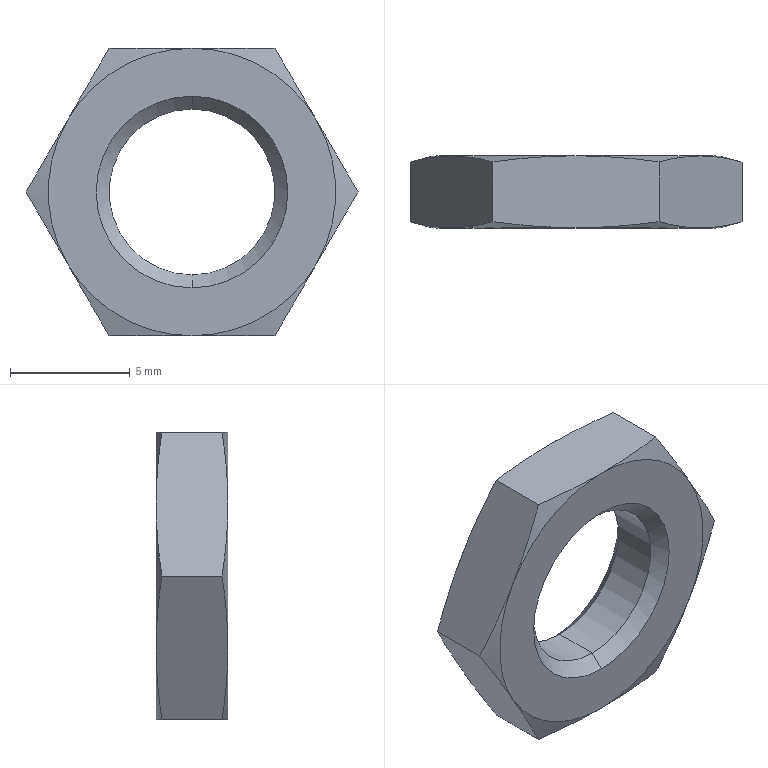Component | SolidWorks | ZPT06UNK6_B5_A80214-1_ZPT2_8_B_NUT0214-1 | 1 solid | 26 faces | box 13.86 x 3 x 12 mm | volume 253 mm3 | cone 16 | plane 8 | cylinder 2 | commonest cylinder face diameters 6.917 x2
build123d program:
from build123d import *

# Parameters (mm, degrees)
CUT_EXTRUDE1_DEPTH      = 1.5
CUT_EXTRUDE1_DEPTH_BACK = 1.5
SKETCH2_R               = 12


with BuildPart() as part:
    # Sketch1 → Revolve1 (revolve)
    with BuildSketch(Plane.XY, mode=Mode.PRIVATE) as revolve1_sk:
        Polygon((3.458, -0.9585), (4, -1.5), (6, -1.5), (9.6, -0.5354), (9.6, 0.5354), (6, 1.5), (4, 1.5), (3.458, 0.9585), align=None)
    revolve(revolve1_sk.sketch.rotate(Axis((0, -1.5, 0), (0, 1, 0)), 270), axis=Axis((0, -1.5, 0), (0, 1, 0)))

    # Sketch2 → Cut-Extrude1 (cut, two sides: drawn at the far end of the back side and taken through both)
    with BuildSketch(Plane(origin=(0, 0, 0), x_dir=(1, 0, 0), z_dir=(0, 1, 0)).offset(-CUT_EXTRUDE1_DEPTH_BACK)):
        Circle(SKETCH2_R)
        Polygon((-6.928, 0), (-3.464, -6), (3.464, -6), (6.928, 0), (3.464, 6), (-3.464, 6), align=None, mode=Mode.SUBTRACT)
    extrude(amount=CUT_EXTRUDE1_DEPTH + CUT_EXTRUDE1_DEPTH_BACK, mode=Mode.SUBTRACT)


solid = part.part

# Placed as in the assembly
solid = solid.moved(Location((-75, -53, 9.1), (0, 0, 0)))
STEP:
#1=CARTESIAN_POINT('',(-2.953,-2.049,0.2221));
#2=VERTEX_POINT('',#1);
#3=CARTESIAN_POINT('',(-2.953,-2.049,0.4944));
#4=VERTEX_POINT('',#3);
#5=CARTESIAN_POINT('',(-2.953,-2.049,0.3583));
#6=DIRECTION('',(0.,1.,0.));
#7=DIRECTION('',(0.,0.,1.));
#8=AXIS2_PLACEMENT_3D('',#5,#6,#7);
#9=CIRCLE('',#8,0.1362);
#10=EDGE_CURVE('',#2,#4,#9,.T.);
#11=ORIENTED_EDGE('',*,*,#10,.F.);
#12=CARTESIAN_POINT('',(-2.953,-2.028,0.2008));
#13=VERTEX_POINT('',#12);
#14=CARTESIAN_POINT('',(-2.953,-2.028,0.2008));
#15=DIRECTION('',(0.,0.7071,-0.7071));
#16=VECTOR('',#15,39.37);
#17=LINE('',#14,#16);
#18=EDGE_CURVE('',#2,#13,#17,.T.);
#19=ORIENTED_EDGE('',*,*,#18,.T.);
#20=CARTESIAN_POINT('',(-2.953,-2.028,0.5157));
#21=VERTEX_POINT('',#20);
#22=CARTESIAN_POINT('',(-2.953,-2.028,0.3583));
#23=DIRECTION('',(0.,1.,0.));
#24=DIRECTION('',(0.,0.,1.));
#25=AXIS2_PLACEMENT_3D('',#22,#23,#24);
#26=CIRCLE('',#25,0.1575);
#27=EDGE_CURVE('',#13,#21,#26,.T.);
#28=ORIENTED_EDGE('',*,*,#27,.T.);
#29=CARTESIAN_POINT('',(-2.953,-2.028,0.5157));
#30=DIRECTION('',(0.,0.7071,0.7071));
#31=VECTOR('',#30,39.37);
#32=LINE('',#29,#31);
#33=EDGE_CURVE('',#4,#21,#32,.T.);
#34=ORIENTED_EDGE('',*,*,#33,.F.);
#35=EDGE_LOOP('',(#11,#19,#28,#34));
#36=FACE_OUTER_BOUND('',#35,.T.);
#37=CARTESIAN_POINT('',(-2.953,-2.028,0.3583));
#38=DIRECTION('',(0.,1.,0.));
#39=DIRECTION('',(0.,0.,1.));
#40=AXIS2_PLACEMENT_3D('',#37,#38,#39);
#41=CONICAL_SURFACE('',#40,0.1575,0.7854);
#42=ADVANCED_FACE('',(#36),#41,.F.);
#43=CARTESIAN_POINT('',(-2.953,-2.124,0.2221));
#44=VERTEX_POINT('',#43);
#45=CARTESIAN_POINT('',(-2.953,-2.124,0.4944));
#46=VERTEX_POINT('',#45);
#47=CARTESIAN_POINT('',(-2.953,-2.124,0.3583));
#48=DIRECTION('',(0.,1.,0.));
#49=DIRECTION('',(0.,0.,1.));
#50=AXIS2_PLACEMENT_3D('',#47,#48,#49);
#51=CIRCLE('',#50,0.1362);
#52=EDGE_CURVE('',#44,#46,#51,.T.);
#53=ORIENTED_EDGE('',*,*,#52,.T.);
#54=CARTESIAN_POINT('',(-2.953,-2.146,0.5157));
#55=VERTEX_POINT('',#54);
#56=CARTESIAN_POINT('',(-2.953,-2.124,0.4944));
#57=DIRECTION('',(0.,-0.7071,0.7071));
#58=VECTOR('',#57,39.37);
#59=LINE('',#56,#58);
#60=EDGE_CURVE('',#46,#55,#59,.T.);
#61=ORIENTED_EDGE('',*,*,#60,.T.);
#62=CARTESIAN_POINT('',(-2.953,-2.146,0.2008));
#63=VERTEX_POINT('',#62);
#64=CARTESIAN_POINT('',(-2.953,-2.146,0.3583));
#65=DIRECTION('',(0.,1.,0.));
#66=DIRECTION('',(0.,0.,1.));
#67=AXIS2_PLACEMENT_3D('',#64,#65,#66);
#68=CIRCLE('',#67,0.1575);
#69=EDGE_CURVE('',#63,#55,#68,.T.);
#70=ORIENTED_EDGE('',*,*,#69,.F.);
#71=CARTESIAN_POINT('',(-2.953,-2.124,0.2221));
#72=DIRECTION('',(0.,-0.7071,-0.7071));
#73=VECTOR('',#72,39.37);
#74=LINE('',#71,#73);
#75=EDGE_CURVE('',#44,#63,#74,.T.);
#76=ORIENTED_EDGE('',*,*,#75,.F.);
#77=EDGE_LOOP('',(#53,#61,#70,#76));
#78=FACE_OUTER_BOUND('',#77,.T.);
#79=CARTESIAN_POINT('',(-2.953,-2.124,0.3583));
#80=DIRECTION('',(0.,-1.,0.));
#81=DIRECTION('',(0.,0.,-1.));
#82=AXIS2_PLACEMENT_3D('',#79,#80,#81);
#83=CONICAL_SURFACE('',#82,0.1362,0.7854);
#84=ADVANCED_FACE('',(#78),#83,.F.);
#85=ORIENTED_EDGE('',*,*,#52,.F.);
#86=CARTESIAN_POINT('',(-2.953,-2.146,0.2221));
#87=DIRECTION('',(0.,1.,0.));
#88=VECTOR('',#87,39.37);
#89=LINE('',#86,#88);
#90=EDGE_CURVE('',#44,#2,#89,.T.);
#91=ORIENTED_EDGE('',*,*,#90,.T.);
#92=ORIENTED_EDGE('',*,*,#10,.T.);
#93=CARTESIAN_POINT('',(-2.953,-2.146,0.4944));
#94=DIRECTION('',(0.,1.,0.));
#95=VECTOR('',#94,39.37);
#96=LINE('',#93,#95);
#97=EDGE_CURVE('',#46,#4,#96,.T.);
#98=ORIENTED_EDGE('',*,*,#97,.F.);
#99=EDGE_LOOP('',(#85,#91,#92,#98));
#100=FACE_OUTER_BOUND('',#99,.T.);
#101=CARTESIAN_POINT('',(-2.953,-2.146,0.3583));
#102=DIRECTION('',(0.,1.,0.));
#103=DIRECTION('',(0.,0.,1.));
#104=AXIS2_PLACEMENT_3D('',#101,#102,#103);
#105=CYLINDRICAL_SURFACE('',#104,0.1362);
#106=ADVANCED_FACE('',(#100),#105,.F.);
#107=CARTESIAN_POINT('',(-2.68,-2.136,0.3583));
#108=VERTEX_POINT('',#107);
#109=CARTESIAN_POINT('',(-2.748,-2.146,0.2402));
#110=VERTEX_POINT('',#109);
#111=CARTESIAN_POINT('',(-2.68,-2.136,0.3583));
#112=CARTESIAN_POINT('',(-2.703,-2.142,0.3189));
#113=CARTESIAN_POINT('',(-2.725,-2.146,0.2795));
#114=CARTESIAN_POINT('',(-2.748,-2.146,0.2402));
#115=B_SPLINE_CURVE_WITH_KNOTS('',3,(#111,#112,#113,#114),.UNSPECIFIED.,.F.,.F.,(4,4),(0.00000023,0.003464),.UNSPECIFIED.);
#116=EDGE_CURVE('',#108,#110,#115,.T.);
#117=ORIENTED_EDGE('',*,*,#116,.F.);
#118=CARTESIAN_POINT('',(-2.748,-2.146,0.4764));
#119=VERTEX_POINT('',#118);
#120=CARTESIAN_POINT('',(-2.748,-2.146,0.4764));
#121=CARTESIAN_POINT('',(-2.725,-2.146,0.437));
#122=CARTESIAN_POINT('',(-2.703,-2.142,0.3976));
#123=CARTESIAN_POINT('',(-2.68,-2.136,0.3583));
#124=B_SPLINE_CURVE_WITH_KNOTS('',3,(#120,#121,#122,#123),.UNSPECIFIED.,.F.,.F.,(4,4),(0.003464,0.006928),.UNSPECIFIED.);
#125=EDGE_CURVE('',#119,#108,#124,.T.);
#126=ORIENTED_EDGE('',*,*,#125,.F.);
#127=CARTESIAN_POINT('',(-2.953,-2.146,0.3583));
#128=DIRECTION('',(0.,1.,0.));
#129=DIRECTION('',(0.,0.,1.));
#130=AXIS2_PLACEMENT_3D('',#127,#128,#129);
#131=CIRCLE('',#130,0.2362);
#132=EDGE_CURVE('',#119,#110,#131,.T.);
#133=ORIENTED_EDGE('',*,*,#132,.T.);
#134=EDGE_LOOP('',(#117,#126,#133));
#135=FACE_OUTER_BOUND('',#134,.T.);
#136=CARTESIAN_POINT('',(-2.953,-2.146,0.3583));
#137=DIRECTION('',(0.,1.,0.));
#138=DIRECTION('',(0.,0.,1.));
#139=AXIS2_PLACEMENT_3D('',#136,#137,#138);
#140=CONICAL_SURFACE('',#139,0.2362,1.309);
#141=ADVANCED_FACE('',(#135),#140,.T.);
#142=CARTESIAN_POINT('',(-2.816,-2.136,0.122));
#143=VERTEX_POINT('',#142);
#144=CARTESIAN_POINT('',(-2.748,-2.146,0.2402));
#145=CARTESIAN_POINT('',(-2.771,-2.146,0.2008));
#146=CARTESIAN_POINT('',(-2.794,-2.142,0.1614));
#147=CARTESIAN_POINT('',(-2.816,-2.136,0.122));
#148=B_SPLINE_CURVE_WITH_KNOTS('',3,(#144,#145,#146,#147),.UNSPECIFIED.,.F.,.F.,(4,4),(0.003464,0.006928),.UNSPECIFIED.);
#149=EDGE_CURVE('',#110,#143,#148,.T.);
#150=ORIENTED_EDGE('',*,*,#149,.F.);
#151=CARTESIAN_POINT('',(-2.953,-2.146,0.122));
#152=VERTEX_POINT('',#151);
#153=CARTESIAN_POINT('',(-2.953,-2.146,0.3583));
#154=DIRECTION('',(0.,1.,0.));
#155=DIRECTION('',(0.,0.,1.));
#156=AXIS2_PLACEMENT_3D('',#153,#154,#155);
#157=CIRCLE('',#156,0.2362);
#158=EDGE_CURVE('',#110,#152,#157,.T.);
#159=ORIENTED_EDGE('',*,*,#158,.T.);
#160=CARTESIAN_POINT('',(-2.816,-2.136,0.122));
#161=CARTESIAN_POINT('',(-2.862,-2.142,0.122));
#162=CARTESIAN_POINT('',(-2.907,-2.146,0.122));
#163=CARTESIAN_POINT('',(-2.953,-2.146,0.122));
#164=B_SPLINE_CURVE_WITH_KNOTS('',3,(#160,#161,#162,#163),.UNSPECIFIED.,.F.,.F.,(4,4),(0.01347,0.01695),.UNSPECIFIED.);
#165=EDGE_CURVE('',#143,#152,#164,.T.);
#166=ORIENTED_EDGE('',*,*,#165,.F.);
#167=EDGE_LOOP('',(#150,#159,#166));
#168=FACE_OUTER_BOUND('',#167,.T.);
#169=CARTESIAN_POINT('',(-2.953,-2.146,0.3583));
#170=DIRECTION('',(0.,1.,0.));
#171=DIRECTION('',(0.,0.,1.));
#172=AXIS2_PLACEMENT_3D('',#169,#170,#171);
#173=CONICAL_SURFACE('',#172,0.2362,1.309);
#174=ADVANCED_FACE('',(#168),#173,.T.);
#175=CARTESIAN_POINT('',(-3.089,-2.136,0.122));
#176=VERTEX_POINT('',#175);
#177=CARTESIAN_POINT('',(-2.953,-2.146,0.122));
#178=CARTESIAN_POINT('',(-2.975,-2.146,0.122));
#179=CARTESIAN_POINT('',(-2.998,-2.145,0.122));
#180=CARTESIAN_POINT('',(-3.044,-2.141,0.122));
#181=CARTESIAN_POINT('',(-3.066,-2.139,0.122));
#182=CARTESIAN_POINT('',(-3.089,-2.136,0.122));
#183=B_SPLINE_CURVE_WITH_KNOTS('',3,(#177,#178,#179,#180,#181,#182),.UNSPECIFIED.,.F.,.F.,(4,2,4),(0.01695,0.01869,0.02043),.UNSPECIFIED.);
#184=EDGE_CURVE('',#152,#176,#183,.T.);
#185=ORIENTED_EDGE('',*,*,#184,.F.);
#186=CARTESIAN_POINT('',(-3.157,-2.146,0.2402));
#187=VERTEX_POINT('',#186);
#188=CARTESIAN_POINT('',(-2.953,-2.146,0.3583));
#189=DIRECTION('',(0.,1.,0.));
#190=DIRECTION('',(0.,0.,1.));
#191=AXIS2_PLACEMENT_3D('',#188,#189,#190);
#192=CIRCLE('',#191,0.2362);
#193=EDGE_CURVE('',#152,#187,#192,.T.);
#194=ORIENTED_EDGE('',*,*,#193,.T.);
#195=CARTESIAN_POINT('',(-3.089,-2.136,0.122));
#196=CARTESIAN_POINT('',(-3.112,-2.142,0.1614));
#197=CARTESIAN_POINT('',(-3.135,-2.146,0.2008));
#198=CARTESIAN_POINT('',(-3.157,-2.146,0.2402));
#199=B_SPLINE_CURVE_WITH_KNOTS('',3,(#195,#196,#197,#198),.UNSPECIFIED.,.F.,.F.,(4,4),(0.00000023,0.003464),.UNSPECIFIED.);
#200=EDGE_CURVE('',#176,#187,#199,.T.);
#201=ORIENTED_EDGE('',*,*,#200,.F.);
#202=EDGE_LOOP('',(#185,#194,#201));
#203=FACE_OUTER_BOUND('',#202,.T.);
#204=CARTESIAN_POINT('',(-2.953,-2.146,0.3583));
#205=DIRECTION('',(0.,1.,0.));
#206=DIRECTION('',(0.,0.,1.));
#207=AXIS2_PLACEMENT_3D('',#204,#205,#206);
#208=CONICAL_SURFACE('',#207,0.2362,1.309);
#209=ADVANCED_FACE('',(#203),#208,.T.);
#210=CARTESIAN_POINT('',(-2.816,-2.136,0.5945));
#211=VERTEX_POINT('',#210);
#212=CARTESIAN_POINT('',(-2.816,-2.136,0.5945));
#213=CARTESIAN_POINT('',(-2.794,-2.142,0.5551));
#214=CARTESIAN_POINT('',(-2.771,-2.146,0.5157));
#215=CARTESIAN_POINT('',(-2.748,-2.146,0.4764));
#216=B_SPLINE_CURVE_WITH_KNOTS('',3,(#212,#213,#214,#215),.UNSPECIFIED.,.F.,.F.,(4,4),(0.00000023,0.003464),.UNSPECIFIED.);
#217=EDGE_CURVE('',#211,#119,#216,.T.);
#218=ORIENTED_EDGE('',*,*,#217,.F.);
#219=CARTESIAN_POINT('',(-2.953,-2.146,0.5945));
#220=VERTEX_POINT('',#219);
#221=CARTESIAN_POINT('',(-2.953,-2.146,0.5945));
#222=CARTESIAN_POINT('',(-2.907,-2.146,0.5945));
#223=CARTESIAN_POINT('',(-2.862,-2.142,0.5945));
#224=CARTESIAN_POINT('',(-2.816,-2.136,0.5945));
#225=B_SPLINE_CURVE_WITH_KNOTS('',3,(#221,#222,#223,#224),.UNSPECIFIED.,.F.,.F.,(4,4),(0.009329,0.01282),.UNSPECIFIED.);
#226=EDGE_CURVE('',#220,#211,#225,.T.);
#227=ORIENTED_EDGE('',*,*,#226,.F.);
#228=CARTESIAN_POINT('',(-2.953,-2.146,0.3583));
#229=DIRECTION('',(0.,1.,0.));
#230=DIRECTION('',(0.,0.,1.));
#231=AXIS2_PLACEMENT_3D('',#228,#229,#230);
#232=CIRCLE('',#231,0.2362);
#233=EDGE_CURVE('',#220,#119,#232,.T.);
#234=ORIENTED_EDGE('',*,*,#233,.T.);
#235=EDGE_LOOP('',(#218,#227,#234));
#236=FACE_OUTER_BOUND('',#235,.T.);
#237=CARTESIAN_POINT('',(-2.953,-2.146,0.3583));
#238=DIRECTION('',(0.,1.,0.));
#239=DIRECTION('',(0.,0.,1.));
#240=AXIS2_PLACEMENT_3D('',#237,#238,#239);
#241=CONICAL_SURFACE('',#240,0.2362,1.309);
#242=ADVANCED_FACE('',(#236),#241,.T.);
#243=CARTESIAN_POINT('',(-3.226,-2.136,0.3583));
#244=VERTEX_POINT('',#243);
#245=CARTESIAN_POINT('',(-3.157,-2.146,0.2402));
#246=CARTESIAN_POINT('',(-3.18,-2.146,0.2795));
#247=CARTESIAN_POINT('',(-3.203,-2.142,0.3189));
#248=CARTESIAN_POINT('',(-3.226,-2.136,0.3583));
#249=B_SPLINE_CURVE_WITH_KNOTS('',3,(#245,#246,#247,#248),.UNSPECIFIED.,.F.,.F.,(4,4),(0.003464,0.006928),.UNSPECIFIED.);
#250=EDGE_CURVE('',#187,#244,#249,.T.);
#251=ORIENTED_EDGE('',*,*,#250,.F.);
#252=CARTESIAN_POINT('',(-3.157,-2.146,0.4764));
#253=VERTEX_POINT('',#252);
#254=CARTESIAN_POINT('',(-2.953,-2.146,0.3583));
#255=DIRECTION('',(0.,1.,0.));
#256=DIRECTION('',(0.,0.,1.));
#257=AXIS2_PLACEMENT_3D('',#254,#255,#256);
#258=CIRCLE('',#257,0.2362);
#259=EDGE_CURVE('',#187,#253,#258,.T.);
#260=ORIENTED_EDGE('',*,*,#259,.T.);
#261=CARTESIAN_POINT('',(-3.226,-2.136,0.3583));
#262=CARTESIAN_POINT('',(-3.203,-2.142,0.3976));
#263=CARTESIAN_POINT('',(-3.18,-2.146,0.437));
#264=CARTESIAN_POINT('',(-3.157,-2.146,0.4764));
#265=B_SPLINE_CURVE_WITH_KNOTS('',3,(#261,#262,#263,#264),.UNSPECIFIED.,.F.,.F.,(4,4),(0.00000023,0.003464),.UNSPECIFIED.);
#266=EDGE_CURVE('',#244,#253,#265,.T.);
#267=ORIENTED_EDGE('',*,*,#266,.F.);
#268=EDGE_LOOP('',(#251,#260,#267));
#269=FACE_OUTER_BOUND('',#268,.T.);
#270=CARTESIAN_POINT('',(-2.953,-2.146,0.3583));
#271=DIRECTION('',(0.,1.,0.));
#272=DIRECTION('',(0.,0.,1.));
#273=AXIS2_PLACEMENT_3D('',#270,#271,#272);
#274=CONICAL_SURFACE('',#273,0.2362,1.309);
#275=ADVANCED_FACE('',(#269),#274,.T.);
#276=CARTESIAN_POINT('',(-3.089,-2.136,0.5945));
#277=VERTEX_POINT('',#276);
#278=CARTESIAN_POINT('',(-3.089,-2.136,0.5945));
#279=CARTESIAN_POINT('',(-3.066,-2.139,0.5945));
#280=CARTESIAN_POINT('',(-3.044,-2.141,0.5945));
#281=CARTESIAN_POINT('',(-2.998,-2.145,0.5945));
#282=CARTESIAN_POINT('',(-2.975,-2.146,0.5945));
#283=CARTESIAN_POINT('',(-2.953,-2.146,0.5945));
#284=B_SPLINE_CURVE_WITH_KNOTS('',3,(#278,#279,#280,#281,#282,#283),.UNSPECIFIED.,.F.,.F.,(4,2,4),(0.005848,0.007589,0.009329),.UNSPECIFIED.);
#285=EDGE_CURVE('',#277,#220,#284,.T.);
#286=ORIENTED_EDGE('',*,*,#285,.F.);
#287=CARTESIAN_POINT('',(-3.157,-2.146,0.4764));
#288=CARTESIAN_POINT('',(-3.135,-2.146,0.5157));
#289=CARTESIAN_POINT('',(-3.112,-2.142,0.5551));
#290=CARTESIAN_POINT('',(-3.089,-2.136,0.5945));
#291=B_SPLINE_CURVE_WITH_KNOTS('',3,(#287,#288,#289,#290),.UNSPECIFIED.,.F.,.F.,(4,4),(0.003464,0.006928),.UNSPECIFIED.);
#292=EDGE_CURVE('',#253,#277,#291,.T.);
#293=ORIENTED_EDGE('',*,*,#292,.F.);
#294=CARTESIAN_POINT('',(-2.953,-2.146,0.3583));
#295=DIRECTION('',(0.,1.,0.));
#296=DIRECTION('',(0.,0.,1.));
#297=AXIS2_PLACEMENT_3D('',#294,#295,#296);
#298=CIRCLE('',#297,0.2362);
#299=EDGE_CURVE('',#253,#220,#298,.T.);
#300=ORIENTED_EDGE('',*,*,#299,.T.);
#301=EDGE_LOOP('',(#286,#293,#300));
#302=FACE_OUTER_BOUND('',#301,.T.);
#303=CARTESIAN_POINT('',(-2.953,-2.146,0.3583));
#304=DIRECTION('',(0.,1.,0.));
#305=DIRECTION('',(0.,0.,1.));
#306=AXIS2_PLACEMENT_3D('',#303,#304,#305);
#307=CONICAL_SURFACE('',#306,0.2362,1.309);
#308=ADVANCED_FACE('',(#302),#307,.T.);
#309=CARTESIAN_POINT('',(-3.226,-2.037,0.3583));
#310=VERTEX_POINT('',#309);
#311=CARTESIAN_POINT('',(-3.157,-2.028,0.2402));
#312=VERTEX_POINT('',#311);
#313=CARTESIAN_POINT('',(-3.226,-2.037,0.3583));
#314=CARTESIAN_POINT('',(-3.203,-2.031,0.3189));
#315=CARTESIAN_POINT('',(-3.18,-2.028,0.2795));
#316=CARTESIAN_POINT('',(-3.157,-2.028,0.2402));
#317=B_SPLINE_CURVE_WITH_KNOTS('',3,(#313,#314,#315,#316),.UNSPECIFIED.,.F.,.F.,(4,4),(0.00000023,0.003464),.UNSPECIFIED.);
#318=EDGE_CURVE('',#310,#312,#317,.T.);
#319=ORIENTED_EDGE('',*,*,#318,.F.);
#320=CARTESIAN_POINT('',(-3.157,-2.028,0.4764));
#321=VERTEX_POINT('',#320);
#322=CARTESIAN_POINT('',(-3.157,-2.028,0.4764));
#323=CARTESIAN_POINT('',(-3.18,-2.028,0.437));
#324=CARTESIAN_POINT('',(-3.203,-2.031,0.3976));
#325=CARTESIAN_POINT('',(-3.226,-2.037,0.3583));
#326=B_SPLINE_CURVE_WITH_KNOTS('',3,(#322,#323,#324,#325),.UNSPECIFIED.,.F.,.F.,(4,4),(0.003464,0.006928),.UNSPECIFIED.);
#327=EDGE_CURVE('',#321,#310,#326,.T.);
#328=ORIENTED_EDGE('',*,*,#327,.F.);
#329=CARTESIAN_POINT('',(-2.953,-2.028,0.3583));
#330=DIRECTION('',(0.,1.,0.));
#331=DIRECTION('',(0.,0.,1.));
#332=AXIS2_PLACEMENT_3D('',#329,#330,#331);
#333=CIRCLE('',#332,0.2362);
#334=EDGE_CURVE('',#312,#321,#333,.T.);
#335=ORIENTED_EDGE('',*,*,#334,.F.);
#336=EDGE_LOOP('',(#319,#328,#335));
#337=FACE_OUTER_BOUND('',#336,.T.);
#338=CARTESIAN_POINT('',(-2.953,-2.066,0.3583));
#339=DIRECTION('',(0.,-1.,0.));
#340=DIRECTION('',(0.,0.,-1.));
#341=AXIS2_PLACEMENT_3D('',#338,#339,#340);
#342=CONICAL_SURFACE('',#341,0.378,1.309);
#343=ADVANCED_FACE('',(#337),#342,.T.);
#344=CARTESIAN_POINT('',(-3.089,-2.037,0.122));
#345=VERTEX_POINT('',#344);
#346=CARTESIAN_POINT('',(-3.157,-2.028,0.2402));
#347=CARTESIAN_POINT('',(-3.135,-2.028,0.2008));
#348=CARTESIAN_POINT('',(-3.112,-2.031,0.1614));
#349=CARTESIAN_POINT('',(-3.089,-2.037,0.122));
#350=B_SPLINE_CURVE_WITH_KNOTS('',3,(#346,#347,#348,#349),.UNSPECIFIED.,.F.,.F.,(4,4),(0.003464,0.006928),.UNSPECIFIED.);
#351=EDGE_CURVE('',#312,#345,#350,.T.);
#352=ORIENTED_EDGE('',*,*,#351,.F.);
#353=CARTESIAN_POINT('',(-2.953,-2.028,0.122));
#354=VERTEX_POINT('',#353);
#355=CARTESIAN_POINT('',(-2.953,-2.028,0.3583));
#356=DIRECTION('',(0.,1.,0.));
#357=DIRECTION('',(0.,0.,1.));
#358=AXIS2_PLACEMENT_3D('',#355,#356,#357);
#359=CIRCLE('',#358,0.2362);
#360=EDGE_CURVE('',#354,#312,#359,.T.);
#361=ORIENTED_EDGE('',*,*,#360,.F.);
#362=CARTESIAN_POINT('',(-3.089,-2.037,0.122));
#363=CARTESIAN_POINT('',(-3.066,-2.034,0.122));
#364=CARTESIAN_POINT('',(-3.044,-2.032,0.122));
#365=CARTESIAN_POINT('',(-2.998,-2.028,0.122));
#366=CARTESIAN_POINT('',(-2.975,-2.028,0.122));
#367=CARTESIAN_POINT('',(-2.953,-2.028,0.122));
#368=B_SPLINE_CURVE_WITH_KNOTS('',3,(#362,#363,#364,#365,#366,#367),.UNSPECIFIED.,.F.,.F.,(4,2,4),(0.005848,0.007589,0.009329),.UNSPECIFIED.);
#369=EDGE_CURVE('',#345,#354,#368,.T.);
#370=ORIENTED_EDGE('',*,*,#369,.F.);
#371=EDGE_LOOP('',(#352,#361,#370));
#372=FACE_OUTER_BOUND('',#371,.T.);
#373=CARTESIAN_POINT('',(-2.953,-2.066,0.3583));
#374=DIRECTION('',(0.,-1.,0.));
#375=DIRECTION('',(0.,0.,-1.));
#376=AXIS2_PLACEMENT_3D('',#373,#374,#375);
#377=CONICAL_SURFACE('',#376,0.378,1.309);
#378=ADVANCED_FACE('',(#372),#377,.T.);
#379=CARTESIAN_POINT('',(-2.816,-2.037,0.122));
#380=VERTEX_POINT('',#379);
#381=CARTESIAN_POINT('',(-2.953,-2.028,0.122));
#382=CARTESIAN_POINT('',(-2.907,-2.028,0.122));
#383=CARTESIAN_POINT('',(-2.862,-2.031,0.122));
#384=CARTESIAN_POINT('',(-2.816,-2.037,0.122));
#385=B_SPLINE_CURVE_WITH_KNOTS('',3,(#381,#382,#383,#384),.UNSPECIFIED.,.F.,.F.,(4,4),(0.009329,0.01282),.UNSPECIFIED.);
#386=EDGE_CURVE('',#354,#380,#385,.T.);
#387=ORIENTED_EDGE('',*,*,#386,.F.);
#388=CARTESIAN_POINT('',(-2.748,-2.028,0.2402));
#389=VERTEX_POINT('',#388);
#390=CARTESIAN_POINT('',(-2.953,-2.028,0.3583));
#391=DIRECTION('',(0.,1.,0.));
#392=DIRECTION('',(0.,0.,1.));
#393=AXIS2_PLACEMENT_3D('',#390,#391,#392);
#394=CIRCLE('',#393,0.2362);
#395=EDGE_CURVE('',#389,#354,#394,.T.);
#396=ORIENTED_EDGE('',*,*,#395,.F.);
#397=CARTESIAN_POINT('',(-2.816,-2.037,0.122));
#398=CARTESIAN_POINT('',(-2.794,-2.031,0.1614));
#399=CARTESIAN_POINT('',(-2.771,-2.028,0.2008));
#400=CARTESIAN_POINT('',(-2.748,-2.028,0.2402));
#401=B_SPLINE_CURVE_WITH_KNOTS('',3,(#397,#398,#399,#400),.UNSPECIFIED.,.F.,.F.,(4,4),(0.00000023,0.003464),.UNSPECIFIED.);
#402=EDGE_CURVE('',#380,#389,#401,.T.);
#403=ORIENTED_EDGE('',*,*,#402,.F.);
#404=EDGE_LOOP('',(#387,#396,#403));
#405=FACE_OUTER_BOUND('',#404,.T.);
#406=CARTESIAN_POINT('',(-2.953,-2.066,0.3583));
#407=DIRECTION('',(0.,-1.,0.));
#408=DIRECTION('',(0.,0.,-1.));
#409=AXIS2_PLACEMENT_3D('',#406,#407,#408);
#410=CONICAL_SURFACE('',#409,0.378,1.309);
#411=ADVANCED_FACE('',(#405),#410,.T.);
#412=CARTESIAN_POINT('',(-2.68,-2.037,0.3583));
#413=VERTEX_POINT('',#412);
#414=CARTESIAN_POINT('',(-2.748,-2.028,0.2402));
#415=CARTESIAN_POINT('',(-2.725,-2.028,0.2795));
#416=CARTESIAN_POINT('',(-2.703,-2.031,0.3189));
#417=CARTESIAN_POINT('',(-2.68,-2.037,0.3583));
#418=B_SPLINE_CURVE_WITH_KNOTS('',3,(#414,#415,#416,#417),.UNSPECIFIED.,.F.,.F.,(4,4),(0.003464,0.006928),.UNSPECIFIED.);
#419=EDGE_CURVE('',#389,#413,#418,.T.);
#420=ORIENTED_EDGE('',*,*,#419,.F.);
#421=CARTESIAN_POINT('',(-2.748,-2.028,0.4764));
#422=VERTEX_POINT('',#421);
#423=CARTESIAN_POINT('',(-2.953,-2.028,0.3583));
#424=DIRECTION('',(0.,1.,0.));
#425=DIRECTION('',(0.,0.,1.));
#426=AXIS2_PLACEMENT_3D('',#423,#424,#425);
#427=CIRCLE('',#426,0.2362);
#428=EDGE_CURVE('',#422,#389,#427,.T.);
#429=ORIENTED_EDGE('',*,*,#428,.F.);
#430=CARTESIAN_POINT('',(-2.68,-2.037,0.3583));
#431=CARTESIAN_POINT('',(-2.703,-2.031,0.3976));
#432=CARTESIAN_POINT('',(-2.725,-2.028,0.437));
#433=CARTESIAN_POINT('',(-2.748,-2.028,0.4764));
#434=B_SPLINE_CURVE_WITH_KNOTS('',3,(#430,#431,#432,#433),.UNSPECIFIED.,.F.,.F.,(4,4),(0.00000023,0.003464),.UNSPECIFIED.);
#435=EDGE_CURVE('',#413,#422,#434,.T.);
#436=ORIENTED_EDGE('',*,*,#435,.F.);
#437=EDGE_LOOP('',(#420,#429,#436));
#438=FACE_OUTER_BOUND('',#437,.T.);
#439=CARTESIAN_POINT('',(-2.953,-2.066,0.3583));
#440=DIRECTION('',(0.,-1.,0.));
#441=DIRECTION('',(0.,0.,-1.));
#442=AXIS2_PLACEMENT_3D('',#439,#440,#441);
#443=CONICAL_SURFACE('',#442,0.378,1.309);
#444=ADVANCED_FACE('',(#438),#443,.T.);
#445=CARTESIAN_POINT('',(-2.816,-2.037,0.5945));
#446=VERTEX_POINT('',#445);
#447=CARTESIAN_POINT('',(-2.748,-2.028,0.4764));
#448=CARTESIAN_POINT('',(-2.771,-2.028,0.5157));
#449=CARTESIAN_POINT('',(-2.794,-2.031,0.5551));
#450=CARTESIAN_POINT('',(-2.816,-2.037,0.5945));
#451=B_SPLINE_CURVE_WITH_KNOTS('',3,(#447,#448,#449,#450),.UNSPECIFIED.,.F.,.F.,(4,4),(0.003464,0.006928),.UNSPECIFIED.);
#452=EDGE_CURVE('',#422,#446,#451,.T.);
#453=ORIENTED_EDGE('',*,*,#452,.F.);
#454=CARTESIAN_POINT('',(-2.953,-2.028,0.5945));
#455=VERTEX_POINT('',#454);
#456=CARTESIAN_POINT('',(-2.953,-2.028,0.3583));
#457=DIRECTION('',(0.,1.,0.));
#458=DIRECTION('',(0.,0.,1.));
#459=AXIS2_PLACEMENT_3D('',#456,#457,#458);
#460=CIRCLE('',#459,0.2362);
#461=EDGE_CURVE('',#455,#422,#460,.T.);
#462=ORIENTED_EDGE('',*,*,#461,.F.);
#463=CARTESIAN_POINT('',(-2.816,-2.037,0.5945));
#464=CARTESIAN_POINT('',(-2.862,-2.031,0.5945));
#465=CARTESIAN_POINT('',(-2.907,-2.028,0.5945));
#466=CARTESIAN_POINT('',(-2.953,-2.028,0.5945));
#467=B_SPLINE_CURVE_WITH_KNOTS('',3,(#463,#464,#465,#466),.UNSPECIFIED.,.F.,.F.,(4,4),(0.01347,0.01695),.UNSPECIFIED.);
#468=EDGE_CURVE('',#446,#455,#467,.T.);
#469=ORIENTED_EDGE('',*,*,#468,.F.);
#470=EDGE_LOOP('',(#453,#462,#469));
#471=FACE_OUTER_BOUND('',#470,.T.);
#472=CARTESIAN_POINT('',(-2.953,-2.066,0.3583));
#473=DIRECTION('',(0.,-1.,0.));
#474=DIRECTION('',(0.,0.,-1.));
#475=AXIS2_PLACEMENT_3D('',#472,#473,#474);
#476=CONICAL_SURFACE('',#475,0.378,1.309);
#477=ADVANCED_FACE('',(#471),#476,.T.);
#478=CARTESIAN_POINT('',(-3.089,-2.037,0.5945));
#479=VERTEX_POINT('',#478);
#480=CARTESIAN_POINT('',(-2.953,-2.028,0.5945));
#481=CARTESIAN_POINT('',(-2.975,-2.028,0.5945));
#482=CARTESIAN_POINT('',(-2.998,-2.028,0.5945));
#483=CARTESIAN_POINT('',(-3.044,-2.032,0.5945));
#484=CARTESIAN_POINT('',(-3.066,-2.034,0.5945));
#485=CARTESIAN_POINT('',(-3.089,-2.037,0.5945));
#486=B_SPLINE_CURVE_WITH_KNOTS('',3,(#480,#481,#482,#483,#484,#485),.UNSPECIFIED.,.F.,.F.,(4,2,4),(0.01695,0.01869,0.02043),.UNSPECIFIED.);
#487=EDGE_CURVE('',#455,#479,#486,.T.);
#488=ORIENTED_EDGE('',*,*,#487,.F.);
#489=CARTESIAN_POINT('',(-2.953,-2.028,0.3583));
#490=DIRECTION('',(0.,1.,0.));
#491=DIRECTION('',(0.,0.,1.));
#492=AXIS2_PLACEMENT_3D('',#489,#490,#491);
#493=CIRCLE('',#492,0.2362);
#494=EDGE_CURVE('',#321,#455,#493,.T.);
#495=ORIENTED_EDGE('',*,*,#494,.F.);
#496=CARTESIAN_POINT('',(-3.089,-2.037,0.5945));
#497=CARTESIAN_POINT('',(-3.112,-2.031,0.5551));
#498=CARTESIAN_POINT('',(-3.135,-2.028,0.5157));
#499=CARTESIAN_POINT('',(-3.157,-2.028,0.4764));
#500=B_SPLINE_CURVE_WITH_KNOTS('',3,(#496,#497,#498,#499),.UNSPECIFIED.,.F.,.F.,(4,4),(0.00000023,0.003464),.UNSPECIFIED.);
#501=EDGE_CURVE('',#479,#321,#500,.T.);
#502=ORIENTED_EDGE('',*,*,#501,.F.);
#503=EDGE_LOOP('',(#488,#495,#502));
#504=FACE_OUTER_BOUND('',#503,.T.);
#505=CARTESIAN_POINT('',(-2.953,-2.066,0.3583));
#506=DIRECTION('',(0.,-1.,0.));
#507=DIRECTION('',(0.,0.,-1.));
#508=AXIS2_PLACEMENT_3D('',#505,#506,#507);
#509=CONICAL_SURFACE('',#508,0.378,1.309);
#510=ADVANCED_FACE('',(#504),#509,.T.);
#511=ORIENTED_EDGE('',*,*,#90,.F.);
#512=CARTESIAN_POINT('',(-2.953,-2.124,0.3583));
#513=DIRECTION('',(0.,1.,0.));
#514=DIRECTION('',(0.,0.,1.));
#515=AXIS2_PLACEMENT_3D('',#512,#513,#514);
#516=CIRCLE('',#515,0.1362);
#517=EDGE_CURVE('',#46,#44,#516,.T.);
#518=ORIENTED_EDGE('',*,*,#517,.F.);
#519=ORIENTED_EDGE('',*,*,#97,.T.);
#520=CARTESIAN_POINT('',(-2.953,-2.049,0.3583));
#521=DIRECTION('',(0.,1.,0.));
#522=DIRECTION('',(0.,0.,1.));
#523=AXIS2_PLACEMENT_3D('',#520,#521,#522);
#524=CIRCLE('',#523,0.1362);
#525=EDGE_CURVE('',#4,#2,#524,.T.);
#526=ORIENTED_EDGE('',*,*,#525,.T.);
#527=EDGE_LOOP('',(#511,#518,#519,#526));
#528=FACE_OUTER_BOUND('',#527,.T.);
#529=CARTESIAN_POINT('',(-2.953,-2.146,0.3583));
#530=DIRECTION('',(0.,1.,0.));
#531=DIRECTION('',(0.,0.,1.));
#532=AXIS2_PLACEMENT_3D('',#529,#530,#531);
#533=CYLINDRICAL_SURFACE('',#532,0.1362);
#534=ADVANCED_FACE('',(#528),#533,.F.);
#535=ORIENTED_EDGE('',*,*,#60,.F.);
#536=ORIENTED_EDGE('',*,*,#517,.T.);
#537=ORIENTED_EDGE('',*,*,#75,.T.);
#538=CARTESIAN_POINT('',(-2.953,-2.146,0.3583));
#539=DIRECTION('',(0.,1.,0.));
#540=DIRECTION('',(0.,0.,1.));
#541=AXIS2_PLACEMENT_3D('',#538,#539,#540);
#542=CIRCLE('',#541,0.1575);
#543=EDGE_CURVE('',#55,#63,#542,.T.);
#544=ORIENTED_EDGE('',*,*,#543,.F.);
#545=EDGE_LOOP('',(#535,#536,#537,#544));
#546=FACE_OUTER_BOUND('',#545,.T.);
#547=CARTESIAN_POINT('',(-2.953,-2.124,0.3583));
#548=DIRECTION('',(0.,-1.,0.));
#549=DIRECTION('',(0.,0.,-1.));
#550=AXIS2_PLACEMENT_3D('',#547,#548,#549);
#551=CONICAL_SURFACE('',#550,0.1362,0.7854);
#552=ADVANCED_FACE('',(#546),#551,.F.);
#553=ORIENTED_EDGE('',*,*,#233,.F.);
#554=ORIENTED_EDGE('',*,*,#299,.F.);
#555=ORIENTED_EDGE('',*,*,#259,.F.);
#556=ORIENTED_EDGE('',*,*,#193,.F.);
#557=ORIENTED_EDGE('',*,*,#158,.F.);
#558=ORIENTED_EDGE('',*,*,#132,.F.);
#559=EDGE_LOOP('',(#553,#554,#555,#556,#557,#558));
#560=FACE_OUTER_BOUND('',#559,.T.);
#561=ORIENTED_EDGE('',*,*,#69,.T.);
#562=ORIENTED_EDGE('',*,*,#543,.T.);
#563=EDGE_LOOP('',(#561,#562));
#564=FACE_BOUND('',#563,.T.);
#565=CARTESIAN_POINT('',(-2.795,-2.146,0.3583));
#566=DIRECTION('',(0.,1.,0.));
#567=DIRECTION('',(0.,0.,1.));
#568=AXIS2_PLACEMENT_3D('',#565,#566,#567);
#569=PLANE('',#568);
#570=ADVANCED_FACE('',(#560,#564),#569,.F.);
#571=CARTESIAN_POINT('',(-2.953,-2.028,0.3583));
#572=DIRECTION('',(0.,1.,0.));
#573=DIRECTION('',(0.,0.,1.));
#574=AXIS2_PLACEMENT_3D('',#571,#572,#573);
#575=CIRCLE('',#574,0.1575);
#576=EDGE_CURVE('',#21,#13,#575,.T.);
#577=ORIENTED_EDGE('',*,*,#576,.F.);
#578=ORIENTED_EDGE('',*,*,#27,.F.);
#579=EDGE_LOOP('',(#577,#578));
#580=FACE_BOUND('',#579,.T.);
#581=ORIENTED_EDGE('',*,*,#461,.T.);
#582=ORIENTED_EDGE('',*,*,#428,.T.);
#583=ORIENTED_EDGE('',*,*,#395,.T.);
#584=ORIENTED_EDGE('',*,*,#360,.T.);
#585=ORIENTED_EDGE('',*,*,#334,.T.);
#586=ORIENTED_EDGE('',*,*,#494,.T.);
#587=EDGE_LOOP('',(#581,#582,#583,#584,#585,#586));
#588=FACE_OUTER_BOUND('',#587,.T.);
#589=CARTESIAN_POINT('',(-2.717,-2.028,0.3583));
#590=DIRECTION('',(0.,-1.,0.));
#591=DIRECTION('',(0.,0.,-1.));
#592=AXIS2_PLACEMENT_3D('',#589,#590,#591);
#593=PLANE('',#592);
#594=ADVANCED_FACE('',(#580,#588),#593,.F.);
#595=ORIENTED_EDGE('',*,*,#18,.F.);
#596=ORIENTED_EDGE('',*,*,#525,.F.);
#597=ORIENTED_EDGE('',*,*,#33,.T.);
#598=ORIENTED_EDGE('',*,*,#576,.T.);
#599=EDGE_LOOP('',(#595,#596,#597,#598));
#600=FACE_OUTER_BOUND('',#599,.T.);
#601=CARTESIAN_POINT('',(-2.953,-2.028,0.3583));
#602=DIRECTION('',(0.,1.,0.));
#603=DIRECTION('',(0.,0.,1.));
#604=AXIS2_PLACEMENT_3D('',#601,#602,#603);
#605=CONICAL_SURFACE('',#604,0.1575,0.7854);
#606=ADVANCED_FACE('',(#600),#605,.F.);
#607=ORIENTED_EDGE('',*,*,#200,.T.);
#608=ORIENTED_EDGE('',*,*,#250,.T.);
#609=CARTESIAN_POINT('',(-3.226,-2.146,0.3583));
#610=DIRECTION('',(0.,1.,0.));
#611=VECTOR('',#610,39.37);
#612=LINE('',#609,#611);
#613=EDGE_CURVE('',#244,#310,#612,.T.);
#614=ORIENTED_EDGE('',*,*,#613,.T.);
#615=ORIENTED_EDGE('',*,*,#318,.T.);
#616=ORIENTED_EDGE('',*,*,#351,.T.);
#617=CARTESIAN_POINT('',(-3.089,-2.146,0.122));
#618=DIRECTION('',(0.,1.,0.));
#619=VECTOR('',#618,39.37);
#620=LINE('',#617,#619);
#621=EDGE_CURVE('',#176,#345,#620,.T.);
#622=ORIENTED_EDGE('',*,*,#621,.F.);
#623=EDGE_LOOP('',(#607,#608,#614,#615,#616,#622));
#624=FACE_OUTER_BOUND('',#623,.T.);
#625=CARTESIAN_POINT('',(-3.089,-2.146,0.122));
#626=DIRECTION('',(-0.866,0.,-0.5));
#627=DIRECTION('',(-0.5,0.,0.866));
#628=AXIS2_PLACEMENT_3D('',#625,#626,#627);
#629=PLANE('',#628);
#630=ADVANCED_FACE('',(#624),#629,.T.);
#631=ORIENTED_EDGE('',*,*,#165,.T.);
#632=ORIENTED_EDGE('',*,*,#184,.T.);
#633=ORIENTED_EDGE('',*,*,#621,.T.);
#634=ORIENTED_EDGE('',*,*,#369,.T.);
#635=ORIENTED_EDGE('',*,*,#386,.T.);
#636=CARTESIAN_POINT('',(-2.816,-2.146,0.122));
#637=DIRECTION('',(0.,1.,0.));
#638=VECTOR('',#637,39.37);
#639=LINE('',#636,#638);
#640=EDGE_CURVE('',#143,#380,#639,.T.);
#641=ORIENTED_EDGE('',*,*,#640,.F.);
#642=EDGE_LOOP('',(#631,#632,#633,#634,#635,#641));
#643=FACE_OUTER_BOUND('',#642,.T.);
#644=CARTESIAN_POINT('',(-2.816,-2.146,0.122));
#645=DIRECTION('',(0.,0.,-1.));
#646=DIRECTION('',(-1.,0.,0.));
#647=AXIS2_PLACEMENT_3D('',#644,#645,#646);
#648=PLANE('',#647);
#649=ADVANCED_FACE('',(#643),#648,.T.);
#650=ORIENTED_EDGE('',*,*,#116,.T.);
#651=ORIENTED_EDGE('',*,*,#149,.T.);
#652=ORIENTED_EDGE('',*,*,#640,.T.);
#653=ORIENTED_EDGE('',*,*,#402,.T.);
#654=ORIENTED_EDGE('',*,*,#419,.T.);
#655=CARTESIAN_POINT('',(-2.68,-2.146,0.3583));
#656=DIRECTION('',(0.,1.,0.));
#657=VECTOR('',#656,39.37);
#658=LINE('',#655,#657);
#659=EDGE_CURVE('',#108,#413,#658,.T.);
#660=ORIENTED_EDGE('',*,*,#659,.F.);
#661=EDGE_LOOP('',(#650,#651,#652,#653,#654,#660));
#662=FACE_OUTER_BOUND('',#661,.T.);
#663=CARTESIAN_POINT('',(-2.68,-2.146,0.3583));
#664=DIRECTION('',(0.866,0.,-0.5));
#665=DIRECTION('',(-0.5,0.,-0.866));
#666=AXIS2_PLACEMENT_3D('',#663,#664,#665);
#667=PLANE('',#666);
#668=ADVANCED_FACE('',(#662),#667,.T.);
#669=ORIENTED_EDGE('',*,*,#217,.T.);
#670=ORIENTED_EDGE('',*,*,#125,.T.);
#671=ORIENTED_EDGE('',*,*,#659,.T.);
#672=ORIENTED_EDGE('',*,*,#435,.T.);
#673=ORIENTED_EDGE('',*,*,#452,.T.);
#674=CARTESIAN_POINT('',(-2.816,-2.146,0.5945));
#675=DIRECTION('',(0.,1.,0.));
#676=VECTOR('',#675,39.37);
#677=LINE('',#674,#676);
#678=EDGE_CURVE('',#211,#446,#677,.T.);
#679=ORIENTED_EDGE('',*,*,#678,.F.);
#680=EDGE_LOOP('',(#669,#670,#671,#672,#673,#679));
#681=FACE_OUTER_BOUND('',#680,.T.);
#682=CARTESIAN_POINT('',(-2.816,-2.146,0.5945));
#683=DIRECTION('',(0.866,0.,0.5));
#684=DIRECTION('',(0.5,0.,-0.866));
#685=AXIS2_PLACEMENT_3D('',#682,#683,#684);
#686=PLANE('',#685);
#687=ADVANCED_FACE('',(#681),#686,.T.);
#688=ORIENTED_EDGE('',*,*,#285,.T.);
#689=ORIENTED_EDGE('',*,*,#226,.T.);
#690=ORIENTED_EDGE('',*,*,#678,.T.);
#691=ORIENTED_EDGE('',*,*,#468,.T.);
#692=ORIENTED_EDGE('',*,*,#487,.T.);
#693=CARTESIAN_POINT('',(-3.089,-2.146,0.5945));
#694=DIRECTION('',(0.,1.,0.));
#695=VECTOR('',#694,39.37);
#696=LINE('',#693,#695);
#697=EDGE_CURVE('',#277,#479,#696,.T.);
#698=ORIENTED_EDGE('',*,*,#697,.F.);
#699=EDGE_LOOP('',(#688,#689,#690,#691,#692,#698));
#700=FACE_OUTER_BOUND('',#699,.T.);
#701=CARTESIAN_POINT('',(-3.089,-2.146,0.5945));
#702=DIRECTION('',(0.,0.,1.));
#703=DIRECTION('',(1.,0.,0.));
#704=AXIS2_PLACEMENT_3D('',#701,#702,#703);
#705=PLANE('',#704);
#706=ADVANCED_FACE('',(#700),#705,.T.);
#707=ORIENTED_EDGE('',*,*,#266,.T.);
#708=ORIENTED_EDGE('',*,*,#292,.T.);
#709=ORIENTED_EDGE('',*,*,#697,.T.);
#710=ORIENTED_EDGE('',*,*,#501,.T.);
#711=ORIENTED_EDGE('',*,*,#327,.T.);
#712=ORIENTED_EDGE('',*,*,#613,.F.);
#713=EDGE_LOOP('',(#707,#708,#709,#710,#711,#712));
#714=FACE_OUTER_BOUND('',#713,.T.);
#715=CARTESIAN_POINT('',(-3.226,-2.146,0.3583));
#716=DIRECTION('',(-0.866,0.,0.5));
#717=DIRECTION('',(0.5,0.,0.866));
#718=AXIS2_PLACEMENT_3D('',#715,#716,#717);
#719=PLANE('',#718);
#720=ADVANCED_FACE('',(#714),#719,.T.);
#721=CLOSED_SHELL('',(#42,#84,#106,#141,#174,#209,#242,#275,#308,#343,#378,#411,#444,#477,#510,#534,#552,#570,#594,#606,#630,#649,#668,#687,#706,#720));
#722=MANIFOLD_SOLID_BREP('',#721);
#723=CARTESIAN_POINT('',(0.,0.,0.));
#724=DIRECTION('',(0.,0.,1.));
#725=DIRECTION('',(1.,0.,0.));
#726=AXIS2_PLACEMENT_3D('',#723,#724,#725);
#727=(LENGTH_UNIT()NAMED_UNIT(*)SI_UNIT($,.METRE.));
#728=LENGTH_MEASURE_WITH_UNIT(LENGTH_MEASURE(0.0254),#727);
#729=DIMENSIONAL_EXPONENTS(1.,0.,0.,0.,0.,0.,0.);
#730=(CONVERSION_BASED_UNIT('',#728)LENGTH_UNIT()NAMED_UNIT(#729));
#731=UNCERTAINTY_MEASURE_WITH_UNIT(LENGTH_MEASURE(0.00001),#730,'','');
#732=(NAMED_UNIT(*)PLANE_ANGLE_UNIT()SI_UNIT($,.RADIAN.));
#733=(NAMED_UNIT(*)SI_UNIT($,.STERADIAN.)SOLID_ANGLE_UNIT());
#734=(GEOMETRIC_REPRESENTATION_CONTEXT(3)GLOBAL_UNCERTAINTY_ASSIGNED_CONTEXT((#731))GLOBAL_UNIT_ASSIGNED_CONTEXT((#730,#732,#733))REPRESENTATION_CONTEXT('',''));
#735=ADVANCED_BREP_SHAPE_REPRESENTATION('',(#722,#726),#734);
#736=COLOUR_RGB('',0.7922,0.8196,0.9333);
#737=FILL_AREA_STYLE_COLOUR('',#736);
#738=FILL_AREA_STYLE('',(#737));
#739=SURFACE_STYLE_FILL_AREA(#738);
#740=SURFACE_SIDE_STYLE('',(#739));
#741=SURFACE_STYLE_USAGE(.BOTH.,#740);
#742=PRESENTATION_STYLE_ASSIGNMENT((#741));
#743=STYLED_ITEM('',(#742),#722);
#744=(LENGTH_UNIT()NAMED_UNIT(*)SI_UNIT($,.METRE.));
#745=LENGTH_MEASURE_WITH_UNIT(LENGTH_MEASURE(0.0254),#744);
#746=DIMENSIONAL_EXPONENTS(1.,0.,0.,0.,0.,0.,0.);
#747=(CONVERSION_BASED_UNIT('',#745)LENGTH_UNIT()NAMED_UNIT(#746));
#748=UNCERTAINTY_MEASURE_WITH_UNIT(LENGTH_MEASURE(0.00001),#747,'','');
#749=(NAMED_UNIT(*)PLANE_ANGLE_UNIT()SI_UNIT($,.RADIAN.));
#750=(NAMED_UNIT(*)SI_UNIT($,.STERADIAN.)SOLID_ANGLE_UNIT());
#751=(GEOMETRIC_REPRESENTATION_CONTEXT(3)GLOBAL_UNCERTAINTY_ASSIGNED_CONTEXT((#748))GLOBAL_UNIT_ASSIGNED_CONTEXT((#747,#749,#750))REPRESENTATION_CONTEXT('',''));
#752=MECHANICAL_DESIGN_GEOMETRIC_PRESENTATION_REPRESENTATION('',(#743),#751);
#753=PRESENTATION_LAYER_ASSIGNMENT('','',(#743));